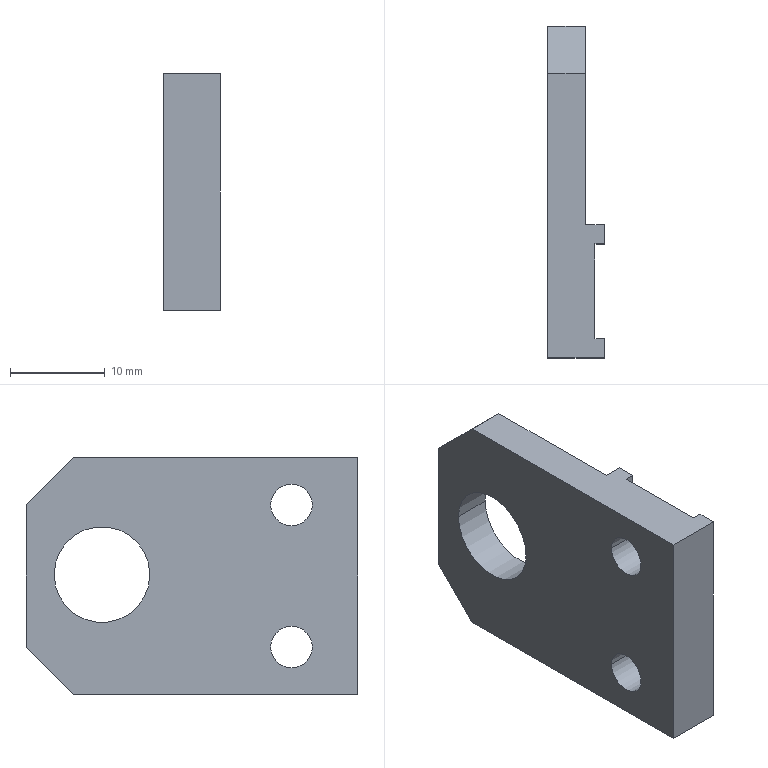Component | SolidWorks | 17268063-1 | 1 solid | 20 faces | box 6 x 35 x 25 mm | volume 3377 mm3 | plane 14 | cylinder 6 | commonest cylinder face diameters 4.4 x4 10.1 x2 | material SKD-11 HRC58° Hard Chrome Plated
build123d program:
from build123d import *

# Parameters (mm, degrees)
SKETCH1_W                  = 25
SKETCH1_H                  = 6
BOSS_EXTRUDE1_DEPTH        = 35
SKETCH2_W                  = 10
SKETCH2_H                  = 1
CUT_EXTRUDE1_DEPTH         = 128.005
SKETCH3_W                  = 21
SKETCH3_H                  = 2
CUT_EXTRUDE2_DEPTH         = 128.005
SKETCH4_R                  = 5.05
CUT_EXTRUDE3_DEPTH         = 49.27
CHAMFER1_SIZE              = 5
F_4_4_4_4_DIAMETER_HOLE1_D = 4.4


with BuildPart() as part:
    # Sketch1 → Boss-Extrude1 (new body)
    with BuildSketch(Plane.XY):
        with Locations((20.5, 116.5)):
            Rectangle(SKETCH1_W, SKETCH1_H)
    extrude(amount=-BOSS_EXTRUDE1_DEPTH)

    # Sketch2 → Cut-Extrude1 (cut, through all)
    with BuildSketch(Plane(origin=(33, 0, 0), x_dir=(0, 0, -1), z_dir=(1, 0, 0))):
        with Locations((7, 114)):
            Rectangle(SKETCH2_W, SKETCH2_H)
    extrude(amount=-CUT_EXTRUDE1_DEPTH, mode=Mode.SUBTRACT)

    # Sketch3 → Cut-Extrude2 (cut, through all)
    with BuildSketch(Plane(origin=(33, 0, 0), x_dir=(0, 0, -1), z_dir=(1, 0, 0))):
        with Locations((24.5, 114.5)):
            Rectangle(SKETCH3_W, SKETCH3_H)
    extrude(amount=-CUT_EXTRUDE2_DEPTH, mode=Mode.SUBTRACT)

    # Sketch4 → Cut-Extrude3 (cut, through all)
    with BuildSketch(Plane.XZ.offset(-115.5)):
        with Locations(Location((20.649, -27, 0), (0, 0, 270))):
            Circle(SKETCH4_R)
    extrude(amount=-CUT_EXTRUDE3_DEPTH, mode=Mode.SUBTRACT)

    # Chamfer1
    chamfer1_edges = [part.edges().sort_by_distance(p)[0] for p in [
        (33, 117.5, -35),
        (8, 117.5, -35),
    ]]
    chamfer(chamfer1_edges, length=CHAMFER1_SIZE)

    # 4.4 _4.4_ Diameter Hole1 (through all)
    with Locations(Plane(origin=(0, 119.5, 0), x_dir=(1, 0, 0), z_dir=(0, 1, 0))):
        with Locations((13, 7), (28, 7)):
            Hole(F_4_4_4_4_DIAMETER_HOLE1_D / 2)


solid = part.part

# Placed as in the assembly
solid = solid.moved(Location((40.5, -54.579, 0.8507), (90, 0, 90)))
STEP:
#1=CARTESIAN_POINT('',(-2.913,-1.787,0.5453));
#2=VERTEX_POINT('',#1);
#3=CARTESIAN_POINT('',(-2.913,-1.96,0.5453));
#4=VERTEX_POINT('',#3);
#5=CARTESIAN_POINT('',(-2.913,-1.873,0.5453));
#6=DIRECTION('',(-1.,0.,0.));
#7=DIRECTION('',(0.,-1.,0.));
#8=AXIS2_PLACEMENT_3D('',#5,#6,#7);
#9=CIRCLE('',#8,0.08661);
#10=EDGE_CURVE('',#2,#4,#9,.T.);
#11=ORIENTED_EDGE('',*,*,#10,.F.);
#12=CARTESIAN_POINT('',(-3.11,-1.787,0.5453));
#13=VERTEX_POINT('',#12);
#14=CARTESIAN_POINT('',(-3.11,-1.787,0.5453));
#15=DIRECTION('',(-1.,0.,0.));
#16=VECTOR('',#15,39.37);
#17=LINE('',#14,#16);
#18=EDGE_CURVE('',#2,#13,#17,.T.);
#19=ORIENTED_EDGE('',*,*,#18,.T.);
#20=CARTESIAN_POINT('',(-3.11,-1.96,0.5453));
#21=VERTEX_POINT('',#20);
#22=CARTESIAN_POINT('',(-3.11,-1.873,0.5453));
#23=DIRECTION('',(-1.,0.,0.));
#24=DIRECTION('',(0.,-1.,0.));
#25=AXIS2_PLACEMENT_3D('',#22,#23,#24);
#26=CIRCLE('',#25,0.08661);
#27=EDGE_CURVE('',#13,#21,#26,.T.);
#28=ORIENTED_EDGE('',*,*,#27,.T.);
#29=CARTESIAN_POINT('',(-3.11,-1.96,0.5453));
#30=DIRECTION('',(-1.,0.,0.));
#31=VECTOR('',#30,39.37);
#32=LINE('',#29,#31);
#33=EDGE_CURVE('',#4,#21,#32,.T.);
#34=ORIENTED_EDGE('',*,*,#33,.F.);
#35=EDGE_LOOP('',(#11,#19,#28,#34));
#36=FACE_OUTER_BOUND('',#35,.T.);
#37=CARTESIAN_POINT('',(-3.11,-1.873,0.5453));
#38=DIRECTION('',(-1.,0.,0.));
#39=DIRECTION('',(0.,-1.,0.));
#40=AXIS2_PLACEMENT_3D('',#37,#38,#39);
#41=CYLINDRICAL_SURFACE('',#40,0.08661);
#42=ADVANCED_FACE('',(#36),#41,.F.);
#43=CARTESIAN_POINT('',(-2.913,-1.787,1.136));
#44=VERTEX_POINT('',#43);
#45=CARTESIAN_POINT('',(-2.913,-1.96,1.136));
#46=VERTEX_POINT('',#45);
#47=CARTESIAN_POINT('',(-2.913,-1.873,1.136));
#48=DIRECTION('',(-1.,0.,0.));
#49=DIRECTION('',(0.,-1.,0.));
#50=AXIS2_PLACEMENT_3D('',#47,#48,#49);
#51=CIRCLE('',#50,0.08661);
#52=EDGE_CURVE('',#44,#46,#51,.T.);
#53=ORIENTED_EDGE('',*,*,#52,.F.);
#54=CARTESIAN_POINT('',(-3.11,-1.787,1.136));
#55=VERTEX_POINT('',#54);
#56=CARTESIAN_POINT('',(-3.11,-1.787,1.136));
#57=DIRECTION('',(-1.,0.,0.));
#58=VECTOR('',#57,39.37);
#59=LINE('',#56,#58);
#60=EDGE_CURVE('',#44,#55,#59,.T.);
#61=ORIENTED_EDGE('',*,*,#60,.T.);
#62=CARTESIAN_POINT('',(-3.11,-1.96,1.136));
#63=VERTEX_POINT('',#62);
#64=CARTESIAN_POINT('',(-3.11,-1.873,1.136));
#65=DIRECTION('',(-1.,0.,0.));
#66=DIRECTION('',(0.,-1.,0.));
#67=AXIS2_PLACEMENT_3D('',#64,#65,#66);
#68=CIRCLE('',#67,0.08661);
#69=EDGE_CURVE('',#55,#63,#68,.T.);
#70=ORIENTED_EDGE('',*,*,#69,.T.);
#71=CARTESIAN_POINT('',(-3.11,-1.96,1.136));
#72=DIRECTION('',(-1.,0.,0.));
#73=VECTOR('',#72,39.37);
#74=LINE('',#71,#73);
#75=EDGE_CURVE('',#46,#63,#74,.T.);
#76=ORIENTED_EDGE('',*,*,#75,.F.);
#77=EDGE_LOOP('',(#53,#61,#70,#76));
#78=FACE_OUTER_BOUND('',#77,.T.);
#79=CARTESIAN_POINT('',(-3.11,-1.873,1.136));
#80=DIRECTION('',(-1.,0.,0.));
#81=DIRECTION('',(0.,-1.,0.));
#82=AXIS2_PLACEMENT_3D('',#79,#80,#81);
#83=CYLINDRICAL_SURFACE('',#82,0.08661);
#84=ADVANCED_FACE('',(#78),#83,.F.);
#85=CARTESIAN_POINT('',(-3.11,-1.285,0.8465));
#86=VERTEX_POINT('',#85);
#87=CARTESIAN_POINT('',(-3.11,-0.887,0.8465));
#88=VERTEX_POINT('',#87);
#89=CARTESIAN_POINT('',(-3.11,-1.086,0.8465));
#90=DIRECTION('',(1.,0.,0.));
#91=DIRECTION('',(0.,1.,0.));
#92=AXIS2_PLACEMENT_3D('',#89,#90,#91);
#93=CIRCLE('',#92,0.1988);
#94=EDGE_CURVE('',#86,#88,#93,.T.);
#95=ORIENTED_EDGE('',*,*,#94,.F.);
#96=CARTESIAN_POINT('',(-2.953,-1.285,0.8465));
#97=VERTEX_POINT('',#96);
#98=CARTESIAN_POINT('',(-3.11,-1.285,0.8465));
#99=DIRECTION('',(1.,0.,0.));
#100=VECTOR('',#99,39.37);
#101=LINE('',#98,#100);
#102=EDGE_CURVE('',#86,#97,#101,.T.);
#103=ORIENTED_EDGE('',*,*,#102,.T.);
#104=CARTESIAN_POINT('',(-2.953,-0.887,0.8465));
#105=VERTEX_POINT('',#104);
#106=CARTESIAN_POINT('',(-2.953,-1.086,0.8465));
#107=DIRECTION('',(1.,0.,0.));
#108=DIRECTION('',(0.,1.,0.));
#109=AXIS2_PLACEMENT_3D('',#106,#107,#108);
#110=CIRCLE('',#109,0.1988);
#111=EDGE_CURVE('',#97,#105,#110,.T.);
#112=ORIENTED_EDGE('',*,*,#111,.T.);
#113=CARTESIAN_POINT('',(-3.11,-0.887,0.8465));
#114=DIRECTION('',(1.,0.,0.));
#115=VECTOR('',#114,39.37);
#116=LINE('',#113,#115);
#117=EDGE_CURVE('',#88,#105,#116,.T.);
#118=ORIENTED_EDGE('',*,*,#117,.F.);
#119=EDGE_LOOP('',(#95,#103,#112,#118));
#120=FACE_OUTER_BOUND('',#119,.T.);
#121=CARTESIAN_POINT('',(-3.11,-1.086,0.8465));
#122=DIRECTION('',(1.,0.,0.));
#123=DIRECTION('',(0.,1.,0.));
#124=AXIS2_PLACEMENT_3D('',#121,#122,#123);
#125=CYLINDRICAL_SURFACE('',#124,0.1988);
#126=ADVANCED_FACE('',(#120),#125,.F.);
#127=CARTESIAN_POINT('',(-2.874,-2.07,0.3485));
#128=VERTEX_POINT('',#127);
#129=CARTESIAN_POINT('',(-2.874,-2.07,1.333));
#130=VERTEX_POINT('',#129);
#131=CARTESIAN_POINT('',(-2.874,-2.07,0.3485));
#132=DIRECTION('',(0.,0.,1.));
#133=VECTOR('',#132,39.37);
#134=LINE('',#131,#133);
#135=EDGE_CURVE('',#128,#130,#134,.T.);
#136=ORIENTED_EDGE('',*,*,#135,.T.);
#137=CARTESIAN_POINT('',(-2.874,-2.149,1.333));
#138=VERTEX_POINT('',#137);
#139=CARTESIAN_POINT('',(-2.874,-0.7708,1.333));
#140=DIRECTION('',(0.,-1.,0.));
#141=VECTOR('',#140,39.37);
#142=LINE('',#139,#141);
#143=EDGE_CURVE('',#130,#138,#142,.T.);
#144=ORIENTED_EDGE('',*,*,#143,.T.);
#145=CARTESIAN_POINT('',(-2.874,-2.149,0.3485));
#146=VERTEX_POINT('',#145);
#147=CARTESIAN_POINT('',(-2.874,-2.149,0.3485));
#148=DIRECTION('',(0.,0.,1.));
#149=VECTOR('',#148,39.37);
#150=LINE('',#147,#149);
#151=EDGE_CURVE('',#146,#138,#150,.T.);
#152=ORIENTED_EDGE('',*,*,#151,.F.);
#153=CARTESIAN_POINT('',(-2.874,-0.7708,0.3485));
#154=DIRECTION('',(0.,-1.,0.));
#155=VECTOR('',#154,39.37);
#156=LINE('',#153,#155);
#157=EDGE_CURVE('',#128,#146,#156,.T.);
#158=ORIENTED_EDGE('',*,*,#157,.F.);
#159=EDGE_LOOP('',(#136,#144,#152,#158));
#160=FACE_OUTER_BOUND('',#159,.T.);
#161=CARTESIAN_POINT('',(-2.874,-0.7708,0.3485));
#162=DIRECTION('',(1.,0.,0.));
#163=DIRECTION('',(0.,1.,0.));
#164=AXIS2_PLACEMENT_3D('',#161,#162,#163);
#165=PLANE('',#164);
#166=ADVANCED_FACE('',(#160),#165,.T.);
#167=CARTESIAN_POINT('',(-3.11,-0.9677,0.3485));
#168=VERTEX_POINT('',#167);
#169=CARTESIAN_POINT('',(-3.11,-2.149,0.3485));
#170=VERTEX_POINT('',#169);
#171=CARTESIAN_POINT('',(-3.11,-0.7708,0.3485));
#172=DIRECTION('',(0.,-1.,0.));
#173=VECTOR('',#172,39.37);
#174=LINE('',#171,#173);
#175=EDGE_CURVE('',#168,#170,#174,.T.);
#176=ORIENTED_EDGE('',*,*,#175,.F.);
#177=CARTESIAN_POINT('',(-2.953,-0.9677,0.3485));
#178=VERTEX_POINT('',#177);
#179=CARTESIAN_POINT('',(-2.953,-0.9677,0.3485));
#180=DIRECTION('',(1.,0.,0.));
#181=VECTOR('',#180,39.37);
#182=LINE('',#179,#181);
#183=EDGE_CURVE('',#168,#178,#182,.T.);
#184=ORIENTED_EDGE('',*,*,#183,.T.);
#185=CARTESIAN_POINT('',(-2.953,-1.598,0.3485));
#186=VERTEX_POINT('',#185);
#187=CARTESIAN_POINT('',(-2.953,-0.7708,0.3485));
#188=DIRECTION('',(0.,-1.,0.));
#189=VECTOR('',#188,39.37);
#190=LINE('',#187,#189);
#191=EDGE_CURVE('',#178,#186,#190,.T.);
#192=ORIENTED_EDGE('',*,*,#191,.T.);
#193=CARTESIAN_POINT('',(-2.874,-1.598,0.3485));
#194=VERTEX_POINT('',#193);
#195=CARTESIAN_POINT('',(-2.874,-1.598,0.3485));
#196=DIRECTION('',(1.,0.,0.));
#197=VECTOR('',#196,39.37);
#198=LINE('',#195,#197);
#199=EDGE_CURVE('',#186,#194,#198,.T.);
#200=ORIENTED_EDGE('',*,*,#199,.T.);
#201=CARTESIAN_POINT('',(-2.874,-1.676,0.3485));
#202=VERTEX_POINT('',#201);
#203=CARTESIAN_POINT('',(-2.874,-0.7708,0.3485));
#204=DIRECTION('',(0.,-1.,0.));
#205=VECTOR('',#204,39.37);
#206=LINE('',#203,#205);
#207=EDGE_CURVE('',#194,#202,#206,.T.);
#208=ORIENTED_EDGE('',*,*,#207,.T.);
#209=CARTESIAN_POINT('',(-2.913,-1.676,0.3485));
#210=VERTEX_POINT('',#209);
#211=CARTESIAN_POINT('',(-2.874,-1.676,0.3485));
#212=DIRECTION('',(-1.,0.,0.));
#213=VECTOR('',#212,39.37);
#214=LINE('',#211,#213);
#215=EDGE_CURVE('',#202,#210,#214,.T.);
#216=ORIENTED_EDGE('',*,*,#215,.T.);
#217=CARTESIAN_POINT('',(-2.913,-2.07,0.3485));
#218=VERTEX_POINT('',#217);
#219=CARTESIAN_POINT('',(-2.913,-2.07,0.3485));
#220=DIRECTION('',(0.,-1.,0.));
#221=VECTOR('',#220,39.37);
#222=LINE('',#219,#221);
#223=EDGE_CURVE('',#210,#218,#222,.T.);
#224=ORIENTED_EDGE('',*,*,#223,.T.);
#225=CARTESIAN_POINT('',(-2.874,-2.07,0.3485));
#226=DIRECTION('',(1.,-0.,0.));
#227=VECTOR('',#226,39.37);
#228=LINE('',#225,#227);
#229=EDGE_CURVE('',#218,#128,#228,.T.);
#230=ORIENTED_EDGE('',*,*,#229,.T.);
#231=ORIENTED_EDGE('',*,*,#157,.T.);
#232=CARTESIAN_POINT('',(-3.11,-2.149,0.3485));
#233=DIRECTION('',(1.,0.,0.));
#234=VECTOR('',#233,39.37);
#235=LINE('',#232,#234);
#236=EDGE_CURVE('',#170,#146,#235,.T.);
#237=ORIENTED_EDGE('',*,*,#236,.F.);
#238=EDGE_LOOP('',(#176,#184,#192,#200,#208,#216,#224,#230,#231,#237));
#239=FACE_OUTER_BOUND('',#238,.T.);
#240=CARTESIAN_POINT('',(-3.11,-0.7708,0.3485));
#241=DIRECTION('',(0.,0.,-1.));
#242=DIRECTION('',(0.,-1.,0.));
#243=AXIS2_PLACEMENT_3D('',#240,#241,#242);
#244=PLANE('',#243);
#245=ADVANCED_FACE('',(#239),#244,.T.);
#246=CARTESIAN_POINT('',(-3.11,-1.873,0.5453));
#247=DIRECTION('',(-1.,0.,0.));
#248=DIRECTION('',(0.,-1.,0.));
#249=AXIS2_PLACEMENT_3D('',#246,#247,#248);
#250=CIRCLE('',#249,0.08661);
#251=EDGE_CURVE('',#21,#13,#250,.T.);
#252=ORIENTED_EDGE('',*,*,#251,.F.);
#253=ORIENTED_EDGE('',*,*,#27,.F.);
#254=EDGE_LOOP('',(#252,#253));
#255=FACE_BOUND('',#254,.T.);
#256=CARTESIAN_POINT('',(-3.11,-1.873,1.136));
#257=DIRECTION('',(-1.,0.,0.));
#258=DIRECTION('',(0.,-1.,0.));
#259=AXIS2_PLACEMENT_3D('',#256,#257,#258);
#260=CIRCLE('',#259,0.08661);
#261=EDGE_CURVE('',#63,#55,#260,.T.);
#262=ORIENTED_EDGE('',*,*,#261,.F.);
#263=ORIENTED_EDGE('',*,*,#69,.F.);
#264=EDGE_LOOP('',(#262,#263));
#265=FACE_BOUND('',#264,.T.);
#266=CARTESIAN_POINT('',(-3.11,-1.086,0.8465));
#267=DIRECTION('',(1.,0.,0.));
#268=DIRECTION('',(0.,1.,0.));
#269=AXIS2_PLACEMENT_3D('',#266,#267,#268);
#270=CIRCLE('',#269,0.1988);
#271=EDGE_CURVE('',#88,#86,#270,.T.);
#272=ORIENTED_EDGE('',*,*,#271,.T.);
#273=ORIENTED_EDGE('',*,*,#94,.T.);
#274=EDGE_LOOP('',(#272,#273));
#275=FACE_BOUND('',#274,.T.);
#276=CARTESIAN_POINT('',(-3.11,-0.7708,1.136));
#277=VERTEX_POINT('',#276);
#278=CARTESIAN_POINT('',(-3.11,-0.7708,0.5453));
#279=VERTEX_POINT('',#278);
#280=CARTESIAN_POINT('',(-3.11,-0.7708,0.3485));
#281=DIRECTION('',(0.,0.,-1.));
#282=VECTOR('',#281,39.37);
#283=LINE('',#280,#282);
#284=EDGE_CURVE('',#277,#279,#283,.T.);
#285=ORIENTED_EDGE('',*,*,#284,.T.);
#286=CARTESIAN_POINT('',(-3.11,-0.8693,0.4469));
#287=DIRECTION('',(0.,-0.7071,-0.7071));
#288=VECTOR('',#287,39.37);
#289=LINE('',#286,#288);
#290=EDGE_CURVE('',#279,#168,#289,.T.);
#291=ORIENTED_EDGE('',*,*,#290,.T.);
#292=ORIENTED_EDGE('',*,*,#175,.T.);
#293=CARTESIAN_POINT('',(-3.11,-2.149,1.333));
#294=VERTEX_POINT('',#293);
#295=CARTESIAN_POINT('',(-3.11,-2.149,0.3485));
#296=DIRECTION('',(0.,0.,-1.));
#297=VECTOR('',#296,39.37);
#298=LINE('',#295,#297);
#299=EDGE_CURVE('',#294,#170,#298,.T.);
#300=ORIENTED_EDGE('',*,*,#299,.F.);
#301=CARTESIAN_POINT('',(-3.11,-0.9677,1.333));
#302=VERTEX_POINT('',#301);
#303=CARTESIAN_POINT('',(-3.11,-0.7708,1.333));
#304=DIRECTION('',(0.,-1.,0.));
#305=VECTOR('',#304,39.37);
#306=LINE('',#303,#305);
#307=EDGE_CURVE('',#302,#294,#306,.T.);
#308=ORIENTED_EDGE('',*,*,#307,.F.);
#309=CARTESIAN_POINT('',(-3.11,-0.3771,0.7422));
#310=DIRECTION('',(0.,0.7071,-0.7071));
#311=VECTOR('',#310,39.37);
#312=LINE('',#309,#311);
#313=EDGE_CURVE('',#302,#277,#312,.T.);
#314=ORIENTED_EDGE('',*,*,#313,.T.);
#315=EDGE_LOOP('',(#285,#291,#292,#300,#308,#314));
#316=FACE_OUTER_BOUND('',#315,.T.);
#317=CARTESIAN_POINT('',(-3.11,-0.7708,0.3485));
#318=DIRECTION('',(-1.,0.,0.));
#319=DIRECTION('',(0.,-1.,0.));
#320=AXIS2_PLACEMENT_3D('',#317,#318,#319);
#321=PLANE('',#320);
#322=ADVANCED_FACE('',(#255,#265,#275,#316),#321,.T.);
#323=CARTESIAN_POINT('',(-2.953,-0.9677,1.333));
#324=VERTEX_POINT('',#323);
#325=CARTESIAN_POINT('',(-2.953,-1.598,1.333));
#326=VERTEX_POINT('',#325);
#327=CARTESIAN_POINT('',(-2.953,-0.7708,1.333));
#328=DIRECTION('',(0.,-1.,0.));
#329=VECTOR('',#328,39.37);
#330=LINE('',#327,#329);
#331=EDGE_CURVE('',#324,#326,#330,.T.);
#332=ORIENTED_EDGE('',*,*,#331,.F.);
#333=CARTESIAN_POINT('',(-3.11,-0.9677,1.333));
#334=DIRECTION('',(-1.,0.,0.));
#335=VECTOR('',#334,39.37);
#336=LINE('',#333,#335);
#337=EDGE_CURVE('',#324,#302,#336,.T.);
#338=ORIENTED_EDGE('',*,*,#337,.T.);
#339=ORIENTED_EDGE('',*,*,#307,.T.);
#340=CARTESIAN_POINT('',(-3.11,-2.149,1.333));
#341=DIRECTION('',(-1.,0.,0.));
#342=VECTOR('',#341,39.37);
#343=LINE('',#340,#342);
#344=EDGE_CURVE('',#138,#294,#343,.T.);
#345=ORIENTED_EDGE('',*,*,#344,.F.);
#346=ORIENTED_EDGE('',*,*,#143,.F.);
#347=CARTESIAN_POINT('',(-2.913,-2.07,1.333));
#348=VERTEX_POINT('',#347);
#349=CARTESIAN_POINT('',(-2.874,-2.07,1.333));
#350=DIRECTION('',(1.,-0.,0.));
#351=VECTOR('',#350,39.37);
#352=LINE('',#349,#351);
#353=EDGE_CURVE('',#348,#130,#352,.T.);
#354=ORIENTED_EDGE('',*,*,#353,.F.);
#355=CARTESIAN_POINT('',(-2.913,-1.676,1.333));
#356=VERTEX_POINT('',#355);
#357=CARTESIAN_POINT('',(-2.913,-2.07,1.333));
#358=DIRECTION('',(0.,-1.,0.));
#359=VECTOR('',#358,39.37);
#360=LINE('',#357,#359);
#361=EDGE_CURVE('',#356,#348,#360,.T.);
#362=ORIENTED_EDGE('',*,*,#361,.F.);
#363=CARTESIAN_POINT('',(-2.874,-1.676,1.333));
#364=VERTEX_POINT('',#363);
#365=CARTESIAN_POINT('',(-2.874,-1.676,1.333));
#366=DIRECTION('',(-1.,0.,0.));
#367=VECTOR('',#366,39.37);
#368=LINE('',#365,#367);
#369=EDGE_CURVE('',#364,#356,#368,.T.);
#370=ORIENTED_EDGE('',*,*,#369,.F.);
#371=CARTESIAN_POINT('',(-2.874,-1.598,1.333));
#372=VERTEX_POINT('',#371);
#373=CARTESIAN_POINT('',(-2.874,-0.7708,1.333));
#374=DIRECTION('',(0.,-1.,0.));
#375=VECTOR('',#374,39.37);
#376=LINE('',#373,#375);
#377=EDGE_CURVE('',#372,#364,#376,.T.);
#378=ORIENTED_EDGE('',*,*,#377,.F.);
#379=CARTESIAN_POINT('',(-2.874,-1.598,1.333));
#380=DIRECTION('',(1.,0.,0.));
#381=VECTOR('',#380,39.37);
#382=LINE('',#379,#381);
#383=EDGE_CURVE('',#326,#372,#382,.T.);
#384=ORIENTED_EDGE('',*,*,#383,.F.);
#385=EDGE_LOOP('',(#332,#338,#339,#345,#346,#354,#362,#370,#378,#384));
#386=FACE_OUTER_BOUND('',#385,.T.);
#387=CARTESIAN_POINT('',(-3.11,-0.7708,1.333));
#388=DIRECTION('',(0.,0.,1.));
#389=DIRECTION('',(0.,1.,0.));
#390=AXIS2_PLACEMENT_3D('',#387,#388,#389);
#391=PLANE('',#390);
#392=ADVANCED_FACE('',(#386),#391,.T.);
#393=CARTESIAN_POINT('',(-2.874,-1.598,0.3485));
#394=DIRECTION('',(0.,0.,1.));
#395=VECTOR('',#394,39.37);
#396=LINE('',#393,#395);
#397=EDGE_CURVE('',#194,#372,#396,.T.);
#398=ORIENTED_EDGE('',*,*,#397,.T.);
#399=ORIENTED_EDGE('',*,*,#377,.T.);
#400=CARTESIAN_POINT('',(-2.874,-1.676,0.3485));
#401=DIRECTION('',(0.,0.,1.));
#402=VECTOR('',#401,39.37);
#403=LINE('',#400,#402);
#404=EDGE_CURVE('',#202,#364,#403,.T.);
#405=ORIENTED_EDGE('',*,*,#404,.F.);
#406=ORIENTED_EDGE('',*,*,#207,.F.);
#407=EDGE_LOOP('',(#398,#399,#405,#406));
#408=FACE_OUTER_BOUND('',#407,.T.);
#409=CARTESIAN_POINT('',(-2.874,-0.7708,0.3485));
#410=DIRECTION('',(1.,0.,0.));
#411=DIRECTION('',(0.,1.,0.));
#412=AXIS2_PLACEMENT_3D('',#409,#410,#411);
#413=PLANE('',#412);
#414=ADVANCED_FACE('',(#408),#413,.T.);
#415=CARTESIAN_POINT('',(-2.953,-0.7708,0.5453));
#416=VERTEX_POINT('',#415);
#417=CARTESIAN_POINT('',(-2.953,-0.7708,1.136));
#418=VERTEX_POINT('',#417);
#419=CARTESIAN_POINT('',(-2.953,-0.7708,0.3485));
#420=DIRECTION('',(0.,0.,1.));
#421=VECTOR('',#420,39.37);
#422=LINE('',#419,#421);
#423=EDGE_CURVE('',#416,#418,#422,.T.);
#424=ORIENTED_EDGE('',*,*,#423,.F.);
#425=CARTESIAN_POINT('',(-3.11,-0.7708,0.5453));
#426=DIRECTION('',(-1.,0.,0.));
#427=VECTOR('',#426,39.37);
#428=LINE('',#425,#427);
#429=EDGE_CURVE('',#416,#279,#428,.T.);
#430=ORIENTED_EDGE('',*,*,#429,.T.);
#431=ORIENTED_EDGE('',*,*,#284,.F.);
#432=CARTESIAN_POINT('',(-2.953,-0.7708,1.136));
#433=DIRECTION('',(1.,0.,0.));
#434=VECTOR('',#433,39.37);
#435=LINE('',#432,#434);
#436=EDGE_CURVE('',#277,#418,#435,.T.);
#437=ORIENTED_EDGE('',*,*,#436,.T.);
#438=EDGE_LOOP('',(#424,#430,#431,#437));
#439=FACE_OUTER_BOUND('',#438,.T.);
#440=CARTESIAN_POINT('',(1.594,-0.7708,0.03349));
#441=DIRECTION('',(0.,-1.,0.));
#442=DIRECTION('',(0.,0.,1.));
#443=AXIS2_PLACEMENT_3D('',#440,#441,#442);
#444=PLANE('',#443);
#445=ADVANCED_FACE('',(#439),#444,.F.);
#446=ORIENTED_EDGE('',*,*,#236,.T.);
#447=ORIENTED_EDGE('',*,*,#151,.T.);
#448=ORIENTED_EDGE('',*,*,#344,.T.);
#449=ORIENTED_EDGE('',*,*,#299,.T.);
#450=EDGE_LOOP('',(#446,#447,#448,#449));
#451=FACE_OUTER_BOUND('',#450,.T.);
#452=CARTESIAN_POINT('',(1.594,-2.149,0.03349));
#453=DIRECTION('',(0.,-1.,0.));
#454=DIRECTION('',(0.,0.,1.));
#455=AXIS2_PLACEMENT_3D('',#452,#453,#454);
#456=PLANE('',#455);
#457=ADVANCED_FACE('',(#451),#456,.T.);
#458=ORIENTED_EDGE('',*,*,#353,.T.);
#459=ORIENTED_EDGE('',*,*,#135,.F.);
#460=ORIENTED_EDGE('',*,*,#229,.F.);
#461=CARTESIAN_POINT('',(-2.913,-2.07,0.3485));
#462=DIRECTION('',(0.,0.,1.));
#463=VECTOR('',#462,39.37);
#464=LINE('',#461,#463);
#465=EDGE_CURVE('',#218,#348,#464,.T.);
#466=ORIENTED_EDGE('',*,*,#465,.T.);
#467=EDGE_LOOP('',(#458,#459,#460,#466));
#468=FACE_OUTER_BOUND('',#467,.T.);
#469=CARTESIAN_POINT('',(-2.874,-2.07,0.3485));
#470=DIRECTION('',(-0.,-1.,0.));
#471=DIRECTION('',(1.,-0.,0.));
#472=AXIS2_PLACEMENT_3D('',#469,#470,#471);
#473=PLANE('',#472);
#474=ADVANCED_FACE('',(#468),#473,.F.);
#475=CARTESIAN_POINT('',(-2.913,-1.873,0.5453));
#476=DIRECTION('',(-1.,0.,0.));
#477=DIRECTION('',(0.,-1.,0.));
#478=AXIS2_PLACEMENT_3D('',#475,#476,#477);
#479=CIRCLE('',#478,0.08661);
#480=EDGE_CURVE('',#4,#2,#479,.T.);
#481=ORIENTED_EDGE('',*,*,#480,.T.);
#482=ORIENTED_EDGE('',*,*,#10,.T.);
#483=EDGE_LOOP('',(#481,#482));
#484=FACE_BOUND('',#483,.T.);
#485=CARTESIAN_POINT('',(-2.913,-1.873,1.136));
#486=DIRECTION('',(-1.,0.,0.));
#487=DIRECTION('',(0.,-1.,0.));
#488=AXIS2_PLACEMENT_3D('',#485,#486,#487);
#489=CIRCLE('',#488,0.08661);
#490=EDGE_CURVE('',#46,#44,#489,.T.);
#491=ORIENTED_EDGE('',*,*,#490,.T.);
#492=ORIENTED_EDGE('',*,*,#52,.T.);
#493=EDGE_LOOP('',(#491,#492));
#494=FACE_BOUND('',#493,.T.);
#495=ORIENTED_EDGE('',*,*,#361,.T.);
#496=ORIENTED_EDGE('',*,*,#465,.F.);
#497=ORIENTED_EDGE('',*,*,#223,.F.);
#498=CARTESIAN_POINT('',(-2.913,-1.676,0.3485));
#499=DIRECTION('',(0.,0.,1.));
#500=VECTOR('',#499,39.37);
#501=LINE('',#498,#500);
#502=EDGE_CURVE('',#210,#356,#501,.T.);
#503=ORIENTED_EDGE('',*,*,#502,.T.);
#504=EDGE_LOOP('',(#495,#496,#497,#503));
#505=FACE_OUTER_BOUND('',#504,.T.);
#506=CARTESIAN_POINT('',(-2.913,-2.07,0.3485));
#507=DIRECTION('',(-1.,0.,0.));
#508=DIRECTION('',(0.,-1.,0.));
#509=AXIS2_PLACEMENT_3D('',#506,#507,#508);
#510=PLANE('',#509);
#511=ADVANCED_FACE('',(#484,#494,#505),#510,.F.);
#512=ORIENTED_EDGE('',*,*,#369,.T.);
#513=ORIENTED_EDGE('',*,*,#502,.F.);
#514=ORIENTED_EDGE('',*,*,#215,.F.);
#515=ORIENTED_EDGE('',*,*,#404,.T.);
#516=EDGE_LOOP('',(#512,#513,#514,#515));
#517=FACE_OUTER_BOUND('',#516,.T.);
#518=CARTESIAN_POINT('',(-2.874,-1.676,0.3485));
#519=DIRECTION('',(0.,1.,0.));
#520=DIRECTION('',(0.,0.,-1.));
#521=AXIS2_PLACEMENT_3D('',#518,#519,#520);
#522=PLANE('',#521);
#523=ADVANCED_FACE('',(#517),#522,.F.);
#524=ORIENTED_EDGE('',*,*,#383,.T.);
#525=ORIENTED_EDGE('',*,*,#397,.F.);
#526=ORIENTED_EDGE('',*,*,#199,.F.);
#527=CARTESIAN_POINT('',(-2.953,-1.598,0.3485));
#528=DIRECTION('',(0.,0.,1.));
#529=VECTOR('',#528,39.37);
#530=LINE('',#527,#529);
#531=EDGE_CURVE('',#186,#326,#530,.T.);
#532=ORIENTED_EDGE('',*,*,#531,.T.);
#533=EDGE_LOOP('',(#524,#525,#526,#532));
#534=FACE_OUTER_BOUND('',#533,.T.);
#535=CARTESIAN_POINT('',(-2.874,-1.598,0.3485));
#536=DIRECTION('',(0.,-1.,0.));
#537=DIRECTION('',(0.,0.,1.));
#538=AXIS2_PLACEMENT_3D('',#535,#536,#537);
#539=PLANE('',#538);
#540=ADVANCED_FACE('',(#534),#539,.F.);
#541=CARTESIAN_POINT('',(-2.953,-1.086,0.8465));
#542=DIRECTION('',(1.,0.,0.));
#543=DIRECTION('',(0.,1.,0.));
#544=AXIS2_PLACEMENT_3D('',#541,#542,#543);
#545=CIRCLE('',#544,0.1988);
#546=EDGE_CURVE('',#105,#97,#545,.T.);
#547=ORIENTED_EDGE('',*,*,#546,.F.);
#548=ORIENTED_EDGE('',*,*,#111,.F.);
#549=EDGE_LOOP('',(#547,#548));
#550=FACE_BOUND('',#549,.T.);
#551=ORIENTED_EDGE('',*,*,#191,.F.);
#552=CARTESIAN_POINT('',(-2.953,-0.9677,0.3485));
#553=DIRECTION('',(0.,0.7071,0.7071));
#554=VECTOR('',#553,39.37);
#555=LINE('',#552,#554);
#556=EDGE_CURVE('',#178,#416,#555,.T.);
#557=ORIENTED_EDGE('',*,*,#556,.T.);
#558=ORIENTED_EDGE('',*,*,#423,.T.);
#559=CARTESIAN_POINT('',(-2.953,-0.9677,1.333));
#560=DIRECTION('',(0.,-0.7071,0.7071));
#561=VECTOR('',#560,39.37);
#562=LINE('',#559,#561);
#563=EDGE_CURVE('',#418,#324,#562,.T.);
#564=ORIENTED_EDGE('',*,*,#563,.T.);
#565=ORIENTED_EDGE('',*,*,#331,.T.);
#566=ORIENTED_EDGE('',*,*,#531,.F.);
#567=EDGE_LOOP('',(#551,#557,#558,#564,#565,#566));
#568=FACE_OUTER_BOUND('',#567,.T.);
#569=CARTESIAN_POINT('',(-2.953,-0.7708,0.3485));
#570=DIRECTION('',(-1.,0.,0.));
#571=DIRECTION('',(0.,-1.,0.));
#572=AXIS2_PLACEMENT_3D('',#569,#570,#571);
#573=PLANE('',#572);
#574=ADVANCED_FACE('',(#550,#568),#573,.F.);
#575=ORIENTED_EDGE('',*,*,#102,.F.);
#576=ORIENTED_EDGE('',*,*,#271,.F.);
#577=ORIENTED_EDGE('',*,*,#117,.T.);
#578=ORIENTED_EDGE('',*,*,#546,.T.);
#579=EDGE_LOOP('',(#575,#576,#577,#578));
#580=FACE_OUTER_BOUND('',#579,.T.);
#581=CARTESIAN_POINT('',(-3.11,-1.086,0.8465));
#582=DIRECTION('',(1.,0.,0.));
#583=DIRECTION('',(0.,1.,0.));
#584=AXIS2_PLACEMENT_3D('',#581,#582,#583);
#585=CYLINDRICAL_SURFACE('',#584,0.1988);
#586=ADVANCED_FACE('',(#580),#585,.F.);
#587=ORIENTED_EDGE('',*,*,#290,.F.);
#588=ORIENTED_EDGE('',*,*,#429,.F.);
#589=ORIENTED_EDGE('',*,*,#556,.F.);
#590=ORIENTED_EDGE('',*,*,#183,.F.);
#591=EDGE_LOOP('',(#587,#588,#589,#590));
#592=FACE_OUTER_BOUND('',#591,.T.);
#593=CARTESIAN_POINT('',(-3.11,-0.9677,0.3485));
#594=DIRECTION('',(0.,0.7071,-0.7071));
#595=DIRECTION('',(-1.,0.,0.));
#596=AXIS2_PLACEMENT_3D('',#593,#594,#595);
#597=PLANE('',#596);
#598=ADVANCED_FACE('',(#592),#597,.T.);
#599=ORIENTED_EDGE('',*,*,#563,.F.);
#600=ORIENTED_EDGE('',*,*,#436,.F.);
#601=ORIENTED_EDGE('',*,*,#313,.F.);
#602=ORIENTED_EDGE('',*,*,#337,.F.);
#603=EDGE_LOOP('',(#599,#600,#601,#602));
#604=FACE_OUTER_BOUND('',#603,.T.);
#605=CARTESIAN_POINT('',(-3.11,-0.9677,1.333));
#606=DIRECTION('',(0.,0.7071,0.7071));
#607=DIRECTION('',(1.,0.,0.));
#608=AXIS2_PLACEMENT_3D('',#605,#606,#607);
#609=PLANE('',#608);
#610=ADVANCED_FACE('',(#604),#609,.T.);
#611=ORIENTED_EDGE('',*,*,#60,.F.);
#612=ORIENTED_EDGE('',*,*,#490,.F.);
#613=ORIENTED_EDGE('',*,*,#75,.T.);
#614=ORIENTED_EDGE('',*,*,#261,.T.);
#615=EDGE_LOOP('',(#611,#612,#613,#614));
#616=FACE_OUTER_BOUND('',#615,.T.);
#617=CARTESIAN_POINT('',(-3.11,-1.873,1.136));
#618=DIRECTION('',(-1.,0.,0.));
#619=DIRECTION('',(0.,-1.,0.));
#620=AXIS2_PLACEMENT_3D('',#617,#618,#619);
#621=CYLINDRICAL_SURFACE('',#620,0.08661);
#622=ADVANCED_FACE('',(#616),#621,.F.);
#623=ORIENTED_EDGE('',*,*,#18,.F.);
#624=ORIENTED_EDGE('',*,*,#480,.F.);
#625=ORIENTED_EDGE('',*,*,#33,.T.);
#626=ORIENTED_EDGE('',*,*,#251,.T.);
#627=EDGE_LOOP('',(#623,#624,#625,#626));
#628=FACE_OUTER_BOUND('',#627,.T.);
#629=CARTESIAN_POINT('',(-3.11,-1.873,0.5453));
#630=DIRECTION('',(-1.,0.,0.));
#631=DIRECTION('',(0.,-1.,0.));
#632=AXIS2_PLACEMENT_3D('',#629,#630,#631);
#633=CYLINDRICAL_SURFACE('',#632,0.08661);
#634=ADVANCED_FACE('',(#628),#633,.F.);
#635=CLOSED_SHELL('',(#42,#84,#126,#166,#245,#322,#392,#414,#445,#457,#474,#511,#523,#540,#574,#586,#598,#610,#622,#634));
#636=MANIFOLD_SOLID_BREP('',#635);
#637=CARTESIAN_POINT('',(0.,0.,0.));
#638=DIRECTION('',(0.,0.,1.));
#639=DIRECTION('',(1.,0.,0.));
#640=AXIS2_PLACEMENT_3D('',#637,#638,#639);
#641=(LENGTH_UNIT()NAMED_UNIT(*)SI_UNIT($,.METRE.));
#642=LENGTH_MEASURE_WITH_UNIT(LENGTH_MEASURE(0.0254),#641);
#643=DIMENSIONAL_EXPONENTS(1.,0.,0.,0.,0.,0.,0.);
#644=(CONVERSION_BASED_UNIT('',#642)LENGTH_UNIT()NAMED_UNIT(#643));
#645=UNCERTAINTY_MEASURE_WITH_UNIT(LENGTH_MEASURE(0.00001),#644,'','');
#646=(NAMED_UNIT(*)PLANE_ANGLE_UNIT()SI_UNIT($,.RADIAN.));
#647=(NAMED_UNIT(*)SI_UNIT($,.STERADIAN.)SOLID_ANGLE_UNIT());
#648=(GEOMETRIC_REPRESENTATION_CONTEXT(3)GLOBAL_UNCERTAINTY_ASSIGNED_CONTEXT((#645))GLOBAL_UNIT_ASSIGNED_CONTEXT((#644,#646,#647))REPRESENTATION_CONTEXT('',''));
#649=ADVANCED_BREP_SHAPE_REPRESENTATION('',(#636,#640),#648);
#650=COLOUR_RGB('',0.7922,0.8196,0.9333);
#651=FILL_AREA_STYLE_COLOUR('',#650);
#652=FILL_AREA_STYLE('',(#651));
#653=SURFACE_STYLE_FILL_AREA(#652);
#654=SURFACE_SIDE_STYLE('',(#653));
#655=SURFACE_STYLE_USAGE(.BOTH.,#654);
#656=PRESENTATION_STYLE_ASSIGNMENT((#655));
#657=STYLED_ITEM('',(#656),#636);
#658=(LENGTH_UNIT()NAMED_UNIT(*)SI_UNIT($,.METRE.));
#659=LENGTH_MEASURE_WITH_UNIT(LENGTH_MEASURE(0.0254),#658);
#660=DIMENSIONAL_EXPONENTS(1.,0.,0.,0.,0.,0.,0.);
#661=(CONVERSION_BASED_UNIT('',#659)LENGTH_UNIT()NAMED_UNIT(#660));
#662=UNCERTAINTY_MEASURE_WITH_UNIT(LENGTH_MEASURE(0.00001),#661,'','');
#663=(NAMED_UNIT(*)PLANE_ANGLE_UNIT()SI_UNIT($,.RADIAN.));
#664=(NAMED_UNIT(*)SI_UNIT($,.STERADIAN.)SOLID_ANGLE_UNIT());
#665=(GEOMETRIC_REPRESENTATION_CONTEXT(3)GLOBAL_UNCERTAINTY_ASSIGNED_CONTEXT((#662))GLOBAL_UNIT_ASSIGNED_CONTEXT((#661,#663,#664))REPRESENTATION_CONTEXT('',''));
#666=MECHANICAL_DESIGN_GEOMETRIC_PRESENTATION_REPRESENTATION('',(#657),#665);
#667=PRESENTATION_LAYER_ASSIGNMENT('','',(#657));